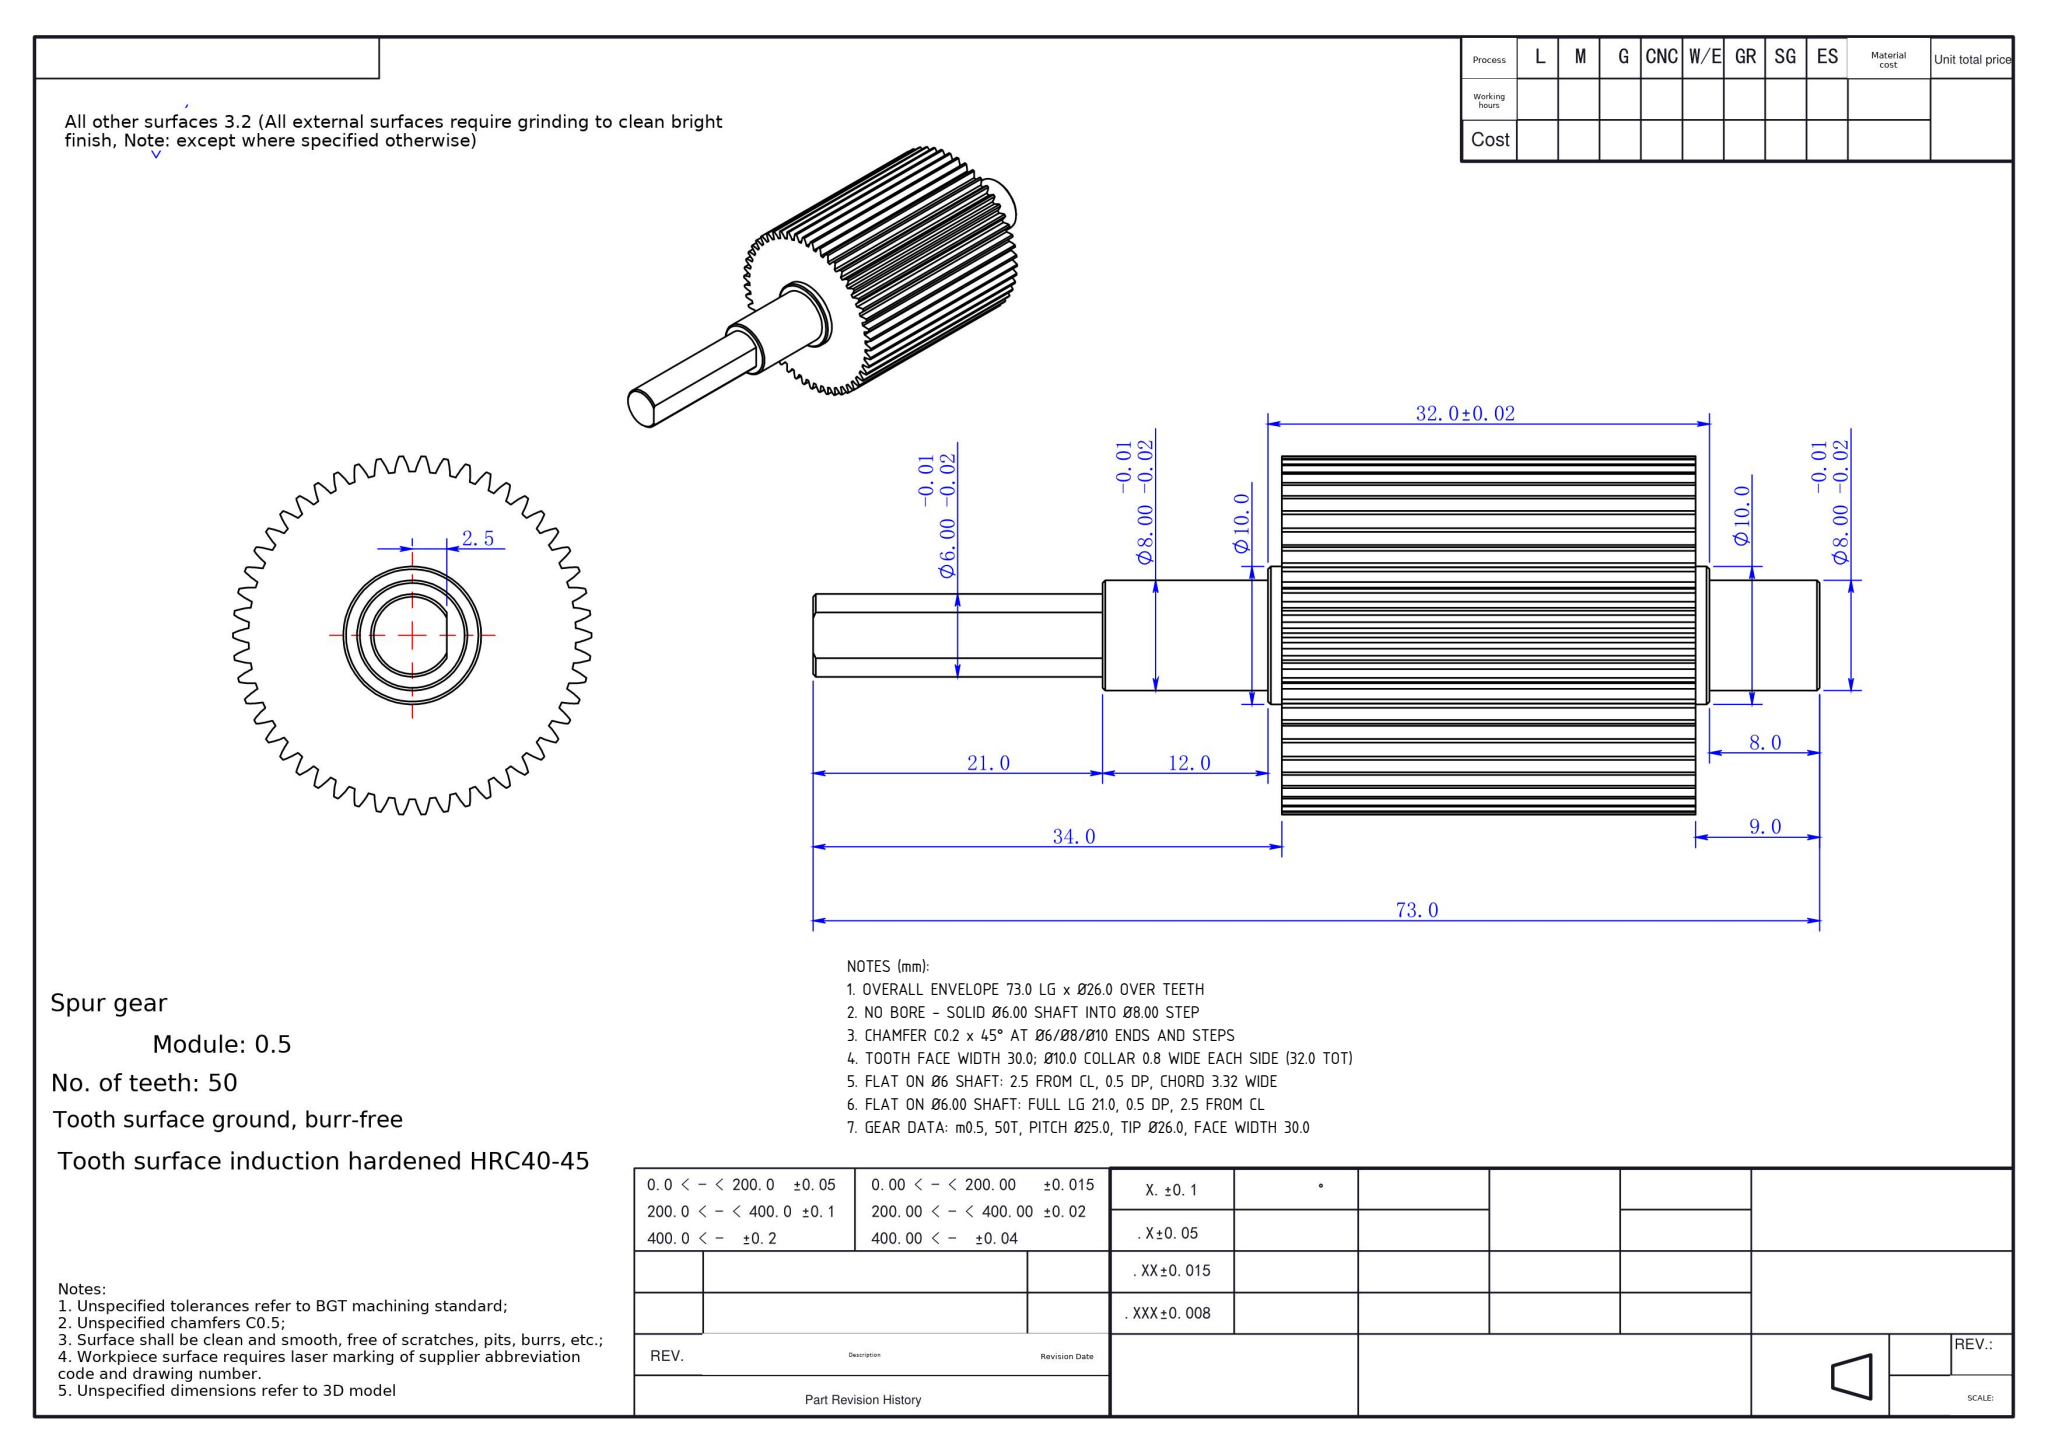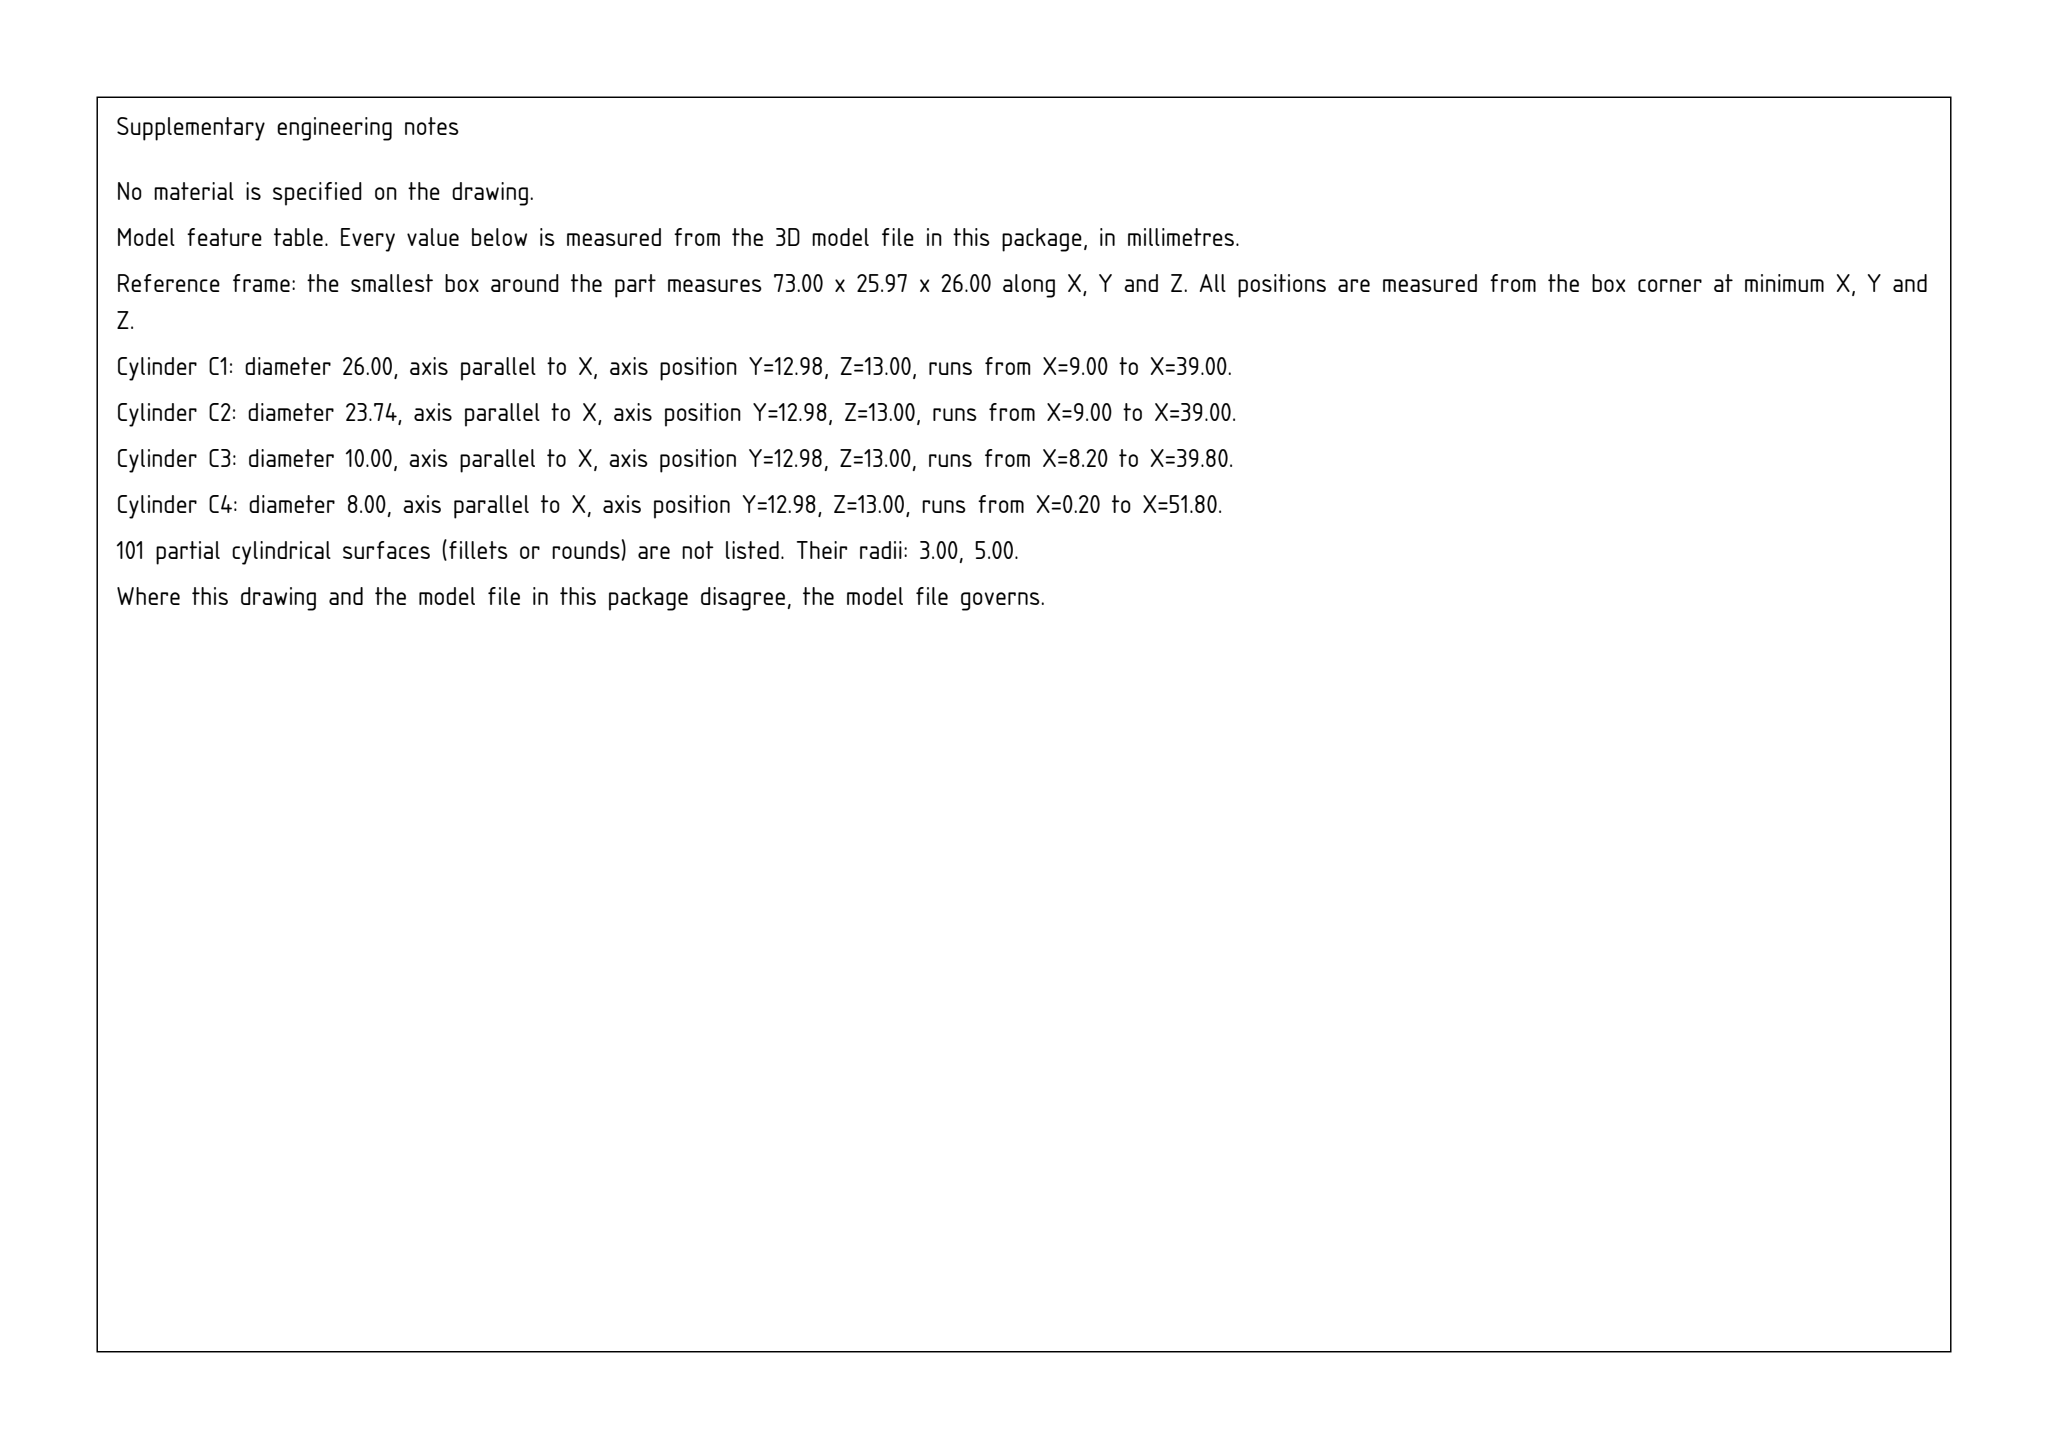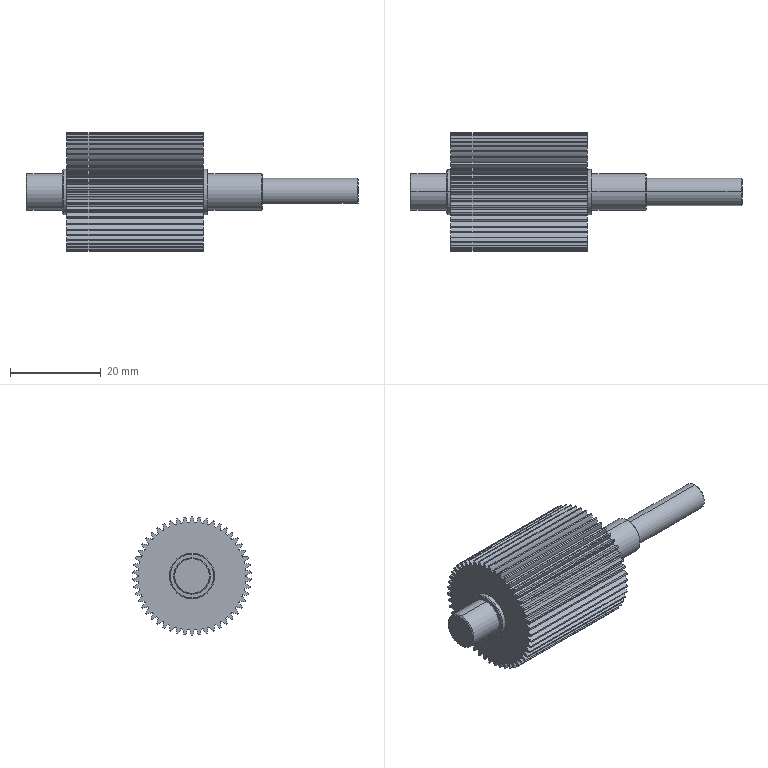Part | SolidWorks | mm | 1 solid | 231 faces | box 73 x 25.97 x 26 mm | volume 16261 mm3 | cylinder 213 | cone 10 | plane 8 | commonest cylinder face diameters 10 x106 26 x51 23.748 x50 8 x4 6 x2
Drawing notes:
OVERALL ENVELOPE 73.0 LG x Ø26.0 OVER TEETH | from the solid: bbox_xyz [73.0, 25.967, 26.0]
NO BORE - SOLID Ø6.00 SHAFT INTO Ø8.00 STEP | from the solid: Only solid cylinders Ø6.00 (L20.8), Ø8.00 (L11.8/7.8), Ø10.0 on x axis; no internal cyl
CHAMFER C0.2 x 45° AT Ø6/Ø8/Ø10 ENDS AND STEPS | from the solid: cones 90° incl angle at ref dia 5.6, 7.6, 9.6 (0.2 off Ø6/Ø8/Ø10)
TOOTH FACE WIDTH 30.0; Ø10.0 COLLAR 0.8 WIDE EACH SIDE (32.0 TOT) | from the solid: tooth cyls L30.0 between x=9 and 39; Ø10.0 L0.8 x4; axis planes x=8,9,39,40
FLAT ON Ø6 SHAFT: 2.5 FROM CL, 0.5 DP, CHORD 3.32 WIDE | from the solid: axis plane [z,10.5] vs Ø6 axis z=13.0 -> 2.5 from CL, 3.0-2.5=0.5 DP, chord 2*sqrt(3²-2.5²)=3.32
FLAT ON Ø6.00 SHAFT: FULL LG 21.0, 0.5 DP, 2.5 FROM CL | from the solid: Plane normal z at offset 10.5 vs shaft axis z=13.0 (0.5 dp, 2.5 from CL); Ø6.00 cyl faces 20.8 lg (21.0 incl C0.2 chamfer, cone 90° ref Ø5.6) span full Ø6 length x52-73
GEAR DATA: m0.5, 50T, PITCH Ø25.0, TIP Ø26.0, FACE WIDTH 30.0 | from the solid: bbox y/z = 25.967/26.0 -> tip Ø26.0; pitch Ø = 0.5 x 50 = 25.0; tooth flank cyls all 30.0 lg between x=9.0 and x=39.0 planes